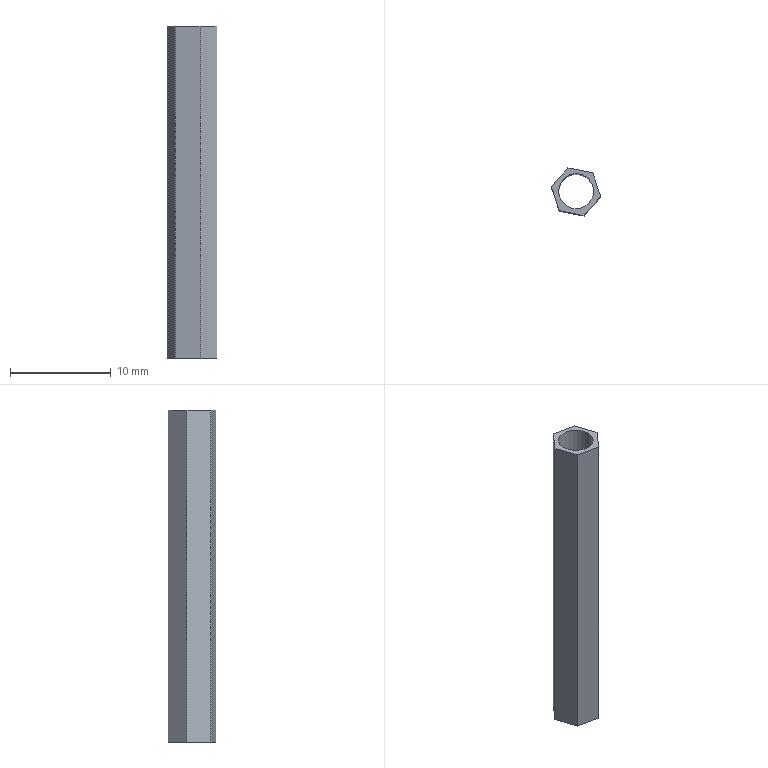Component | SolidWorks | HexStandoff-2 | 1 solid | 10 faces | box 4.92 x 4.75 x 33 mm | volume 227 mm3 | plane 8 | cylinder 2 | commonest cylinder face diameters 3.47 x2
build123d program:
from build123d import *

# Parameters (mm, degrees)
BOSS_EXTRUDE1_DEPTH     = 33
CUT_EXTRUDE1_DEPTH      = 164.264
CUT_EXTRUDE1_DEPTH_BACK = 164.264
SKETCH2_R               = 1.735


with BuildPart() as part:
    # Sketch1 → Boss-Extrude1 (new body)
    with BuildSketch(Plane.XY):
        Polygon((-154.452, -21.596), (-156.91, -22.094), (-157.708, -24.471), (-156.048, -26.351), (-153.59, -25.853), (-152.792, -23.476), align=None)
    extrude(amount=BOSS_EXTRUDE1_DEPTH)

    # Sketch2 → Cut-Extrude1 (cut, two sides: drawn at the far end of the back side and taken through both)
    with BuildSketch(Plane.XY.offset(33).offset(-CUT_EXTRUDE1_DEPTH_BACK)):
        with Locations((-155.258, -23.933)):
            Circle(SKETCH2_R)
    extrude(amount=CUT_EXTRUDE1_DEPTH + CUT_EXTRUDE1_DEPTH_BACK, mode=Mode.SUBTRACT)


solid = part.part

# Placed as in the assembly
solid = solid.moved(Location((-60.744, 0.3563, 17.5), (-180, 0, 180)))
STEP:
#1=COLOUR_RGB('',0.7922,0.8196,0.9333);
#2=FILL_AREA_STYLE_COLOUR('',#1);
#3=FILL_AREA_STYLE('',(#2));
#4=SURFACE_STYLE_FILL_AREA(#3);
#5=SURFACE_SIDE_STYLE('',(#4));
#6=SURFACE_STYLE_USAGE(.BOTH.,#5);
#7=PRESENTATION_STYLE_ASSIGNMENT((#6));
#8=CARTESIAN_POINT('',(3.789,-0.9282,0.689));
#9=VERTEX_POINT('',#8);
#10=CARTESIAN_POINT('',(3.653,-0.9282,0.689));
#11=VERTEX_POINT('',#10);
#12=CARTESIAN_POINT('',(3.721,-0.9282,0.689));
#13=DIRECTION('',(0.,0.,-1.));
#14=DIRECTION('',(-1.,0.,0.));
#15=AXIS2_PLACEMENT_3D('',#12,#13,#14);
#16=CIRCLE('',#15,0.06831);
#17=EDGE_CURVE('',#9,#11,#16,.T.);
#18=ORIENTED_EDGE('',*,*,#17,.F.);
#19=CARTESIAN_POINT('',(3.789,-0.9282,-0.6102));
#20=VERTEX_POINT('',#19);
#21=CARTESIAN_POINT('',(3.789,-0.9282,0.689));
#22=DIRECTION('',(0.,0.,-1.));
#23=VECTOR('',#22,39.37);
#24=LINE('',#21,#23);
#25=EDGE_CURVE('',#9,#20,#24,.T.);
#26=ORIENTED_EDGE('',*,*,#25,.T.);
#27=CARTESIAN_POINT('',(3.653,-0.9282,-0.6102));
#28=VERTEX_POINT('',#27);
#29=CARTESIAN_POINT('',(3.721,-0.9282,-0.6102));
#30=DIRECTION('',(0.,0.,-1.));
#31=DIRECTION('',(-1.,0.,0.));
#32=AXIS2_PLACEMENT_3D('',#29,#30,#31);
#33=CIRCLE('',#32,0.06831);
#34=EDGE_CURVE('',#20,#28,#33,.T.);
#35=ORIENTED_EDGE('',*,*,#34,.T.);
#36=CARTESIAN_POINT('',(3.653,-0.9282,0.689));
#37=DIRECTION('',(0.,0.,-1.));
#38=VECTOR('',#37,39.37);
#39=LINE('',#36,#38);
#40=EDGE_CURVE('',#11,#28,#39,.T.);
#41=ORIENTED_EDGE('',*,*,#40,.F.);
#42=EDGE_LOOP('',(#18,#26,#35,#41));
#43=FACE_OUTER_BOUND('',#42,.T.);
#44=CARTESIAN_POINT('',(3.721,-0.9282,0.689));
#45=DIRECTION('',(0.,0.,-1.));
#46=DIRECTION('',(-1.,0.,0.));
#47=AXIS2_PLACEMENT_3D('',#44,#45,#46);
#48=CYLINDRICAL_SURFACE('',#47,0.06831);
#49=ADVANCED_FACE('',(#43),#48,.F.);
#50=CARTESIAN_POINT('',(3.624,-0.9102,0.689));
#51=VERTEX_POINT('',#50);
#52=CARTESIAN_POINT('',(3.689,-0.8362,0.689));
#53=VERTEX_POINT('',#52);
#54=CARTESIAN_POINT('',(3.624,-0.9102,0.689));
#55=DIRECTION('',(0.6619,0.7496,0.));
#56=VECTOR('',#55,39.37);
#57=LINE('',#54,#56);
#58=EDGE_CURVE('',#51,#53,#57,.T.);
#59=ORIENTED_EDGE('',*,*,#58,.T.);
#60=CARTESIAN_POINT('',(3.689,-0.8362,-0.6102));
#61=VERTEX_POINT('',#60);
#62=CARTESIAN_POINT('',(3.689,-0.8362,-0.6102));
#63=DIRECTION('',(0.,0.,1.));
#64=VECTOR('',#63,39.37);
#65=LINE('',#62,#64);
#66=EDGE_CURVE('',#61,#53,#65,.T.);
#67=ORIENTED_EDGE('',*,*,#66,.F.);
#68=CARTESIAN_POINT('',(3.624,-0.9102,-0.6102));
#69=VERTEX_POINT('',#68);
#70=CARTESIAN_POINT('',(3.624,-0.9102,-0.6102));
#71=DIRECTION('',(0.6619,0.7496,0.));
#72=VECTOR('',#71,39.37);
#73=LINE('',#70,#72);
#74=EDGE_CURVE('',#69,#61,#73,.T.);
#75=ORIENTED_EDGE('',*,*,#74,.F.);
#76=CARTESIAN_POINT('',(3.624,-0.9102,-0.6102));
#77=DIRECTION('',(0.,0.,1.));
#78=VECTOR('',#77,39.37);
#79=LINE('',#76,#78);
#80=EDGE_CURVE('',#69,#51,#79,.T.);
#81=ORIENTED_EDGE('',*,*,#80,.T.);
#82=EDGE_LOOP('',(#59,#67,#75,#81));
#83=FACE_OUTER_BOUND('',#82,.T.);
#84=CARTESIAN_POINT('',(3.624,-0.9102,-0.6102));
#85=DIRECTION('',(0.7496,-0.6619,0.));
#86=DIRECTION('',(-0.6619,-0.7496,0.));
#87=AXIS2_PLACEMENT_3D('',#84,#85,#86);
#88=PLANE('',#87);
#89=ADVANCED_FACE('',(#83),#88,.F.);
#90=CARTESIAN_POINT('',(3.786,-0.8558,0.689));
#91=VERTEX_POINT('',#90);
#92=CARTESIAN_POINT('',(3.689,-0.8362,0.689));
#93=DIRECTION('',(0.9801,-0.1985,0.));
#94=VECTOR('',#93,39.37);
#95=LINE('',#92,#94);
#96=EDGE_CURVE('',#53,#91,#95,.T.);
#97=ORIENTED_EDGE('',*,*,#96,.T.);
#98=CARTESIAN_POINT('',(3.786,-0.8558,-0.6102));
#99=VERTEX_POINT('',#98);
#100=CARTESIAN_POINT('',(3.786,-0.8558,-0.6102));
#101=DIRECTION('',(0.,0.,1.));
#102=VECTOR('',#101,39.37);
#103=LINE('',#100,#102);
#104=EDGE_CURVE('',#99,#91,#103,.T.);
#105=ORIENTED_EDGE('',*,*,#104,.F.);
#106=CARTESIAN_POINT('',(3.689,-0.8362,-0.6102));
#107=DIRECTION('',(0.9801,-0.1985,0.));
#108=VECTOR('',#107,39.37);
#109=LINE('',#106,#108);
#110=EDGE_CURVE('',#61,#99,#109,.T.);
#111=ORIENTED_EDGE('',*,*,#110,.F.);
#112=ORIENTED_EDGE('',*,*,#66,.T.);
#113=EDGE_LOOP('',(#97,#105,#111,#112));
#114=FACE_OUTER_BOUND('',#113,.T.);
#115=CARTESIAN_POINT('',(3.689,-0.8362,-0.6102));
#116=DIRECTION('',(-0.1985,-0.9801,0.));
#117=DIRECTION('',(-0.9801,0.1985,0.));
#118=AXIS2_PLACEMENT_3D('',#115,#116,#117);
#119=PLANE('',#118);
#120=ADVANCED_FACE('',(#114),#119,.F.);
#121=CARTESIAN_POINT('',(3.817,-0.9494,0.689));
#122=VERTEX_POINT('',#121);
#123=CARTESIAN_POINT('',(3.786,-0.8558,0.689));
#124=DIRECTION('',(0.3182,-0.948,0.));
#125=VECTOR('',#124,39.37);
#126=LINE('',#123,#125);
#127=EDGE_CURVE('',#91,#122,#126,.T.);
#128=ORIENTED_EDGE('',*,*,#127,.T.);
#129=CARTESIAN_POINT('',(3.817,-0.9494,-0.6102));
#130=VERTEX_POINT('',#129);
#131=CARTESIAN_POINT('',(3.817,-0.9494,-0.6102));
#132=DIRECTION('',(0.,0.,1.));
#133=VECTOR('',#132,39.37);
#134=LINE('',#131,#133);
#135=EDGE_CURVE('',#130,#122,#134,.T.);
#136=ORIENTED_EDGE('',*,*,#135,.F.);
#137=CARTESIAN_POINT('',(3.786,-0.8558,-0.6102));
#138=DIRECTION('',(0.3182,-0.948,0.));
#139=VECTOR('',#138,39.37);
#140=LINE('',#137,#139);
#141=EDGE_CURVE('',#99,#130,#140,.T.);
#142=ORIENTED_EDGE('',*,*,#141,.F.);
#143=ORIENTED_EDGE('',*,*,#104,.T.);
#144=EDGE_LOOP('',(#128,#136,#142,#143));
#145=FACE_OUTER_BOUND('',#144,.T.);
#146=CARTESIAN_POINT('',(3.786,-0.8558,-0.6102));
#147=DIRECTION('',(-0.948,-0.3182,0.));
#148=DIRECTION('',(-0.3182,0.948,0.));
#149=AXIS2_PLACEMENT_3D('',#146,#147,#148);
#150=PLANE('',#149);
#151=ADVANCED_FACE('',(#145),#150,.F.);
#152=CARTESIAN_POINT('',(3.752,-1.023,0.689));
#153=VERTEX_POINT('',#152);
#154=CARTESIAN_POINT('',(3.817,-0.9494,0.689));
#155=DIRECTION('',(-0.6619,-0.7496,0.));
#156=VECTOR('',#155,39.37);
#157=LINE('',#154,#156);
#158=EDGE_CURVE('',#122,#153,#157,.T.);
#159=ORIENTED_EDGE('',*,*,#158,.T.);
#160=CARTESIAN_POINT('',(3.752,-1.023,-0.6102));
#161=VERTEX_POINT('',#160);
#162=CARTESIAN_POINT('',(3.752,-1.023,-0.6102));
#163=DIRECTION('',(0.,0.,1.));
#164=VECTOR('',#163,39.37);
#165=LINE('',#162,#164);
#166=EDGE_CURVE('',#161,#153,#165,.T.);
#167=ORIENTED_EDGE('',*,*,#166,.F.);
#168=CARTESIAN_POINT('',(3.817,-0.9494,-0.6102));
#169=DIRECTION('',(-0.6619,-0.7496,0.));
#170=VECTOR('',#169,39.37);
#171=LINE('',#168,#170);
#172=EDGE_CURVE('',#130,#161,#171,.T.);
#173=ORIENTED_EDGE('',*,*,#172,.F.);
#174=ORIENTED_EDGE('',*,*,#135,.T.);
#175=EDGE_LOOP('',(#159,#167,#173,#174));
#176=FACE_OUTER_BOUND('',#175,.T.);
#177=CARTESIAN_POINT('',(3.817,-0.9494,-0.6102));
#178=DIRECTION('',(-0.7496,0.6619,0.));
#179=DIRECTION('',(0.6619,0.7496,0.));
#180=AXIS2_PLACEMENT_3D('',#177,#178,#179);
#181=PLANE('',#180);
#182=ADVANCED_FACE('',(#176),#181,.F.);
#183=CARTESIAN_POINT('',(3.655,-1.004,0.689));
#184=VERTEX_POINT('',#183);
#185=CARTESIAN_POINT('',(3.752,-1.023,0.689));
#186=DIRECTION('',(-0.9801,0.1985,0.));
#187=VECTOR('',#186,39.37);
#188=LINE('',#185,#187);
#189=EDGE_CURVE('',#153,#184,#188,.T.);
#190=ORIENTED_EDGE('',*,*,#189,.T.);
#191=CARTESIAN_POINT('',(3.655,-1.004,-0.6102));
#192=VERTEX_POINT('',#191);
#193=CARTESIAN_POINT('',(3.655,-1.004,-0.6102));
#194=DIRECTION('',(0.,0.,1.));
#195=VECTOR('',#194,39.37);
#196=LINE('',#193,#195);
#197=EDGE_CURVE('',#192,#184,#196,.T.);
#198=ORIENTED_EDGE('',*,*,#197,.F.);
#199=CARTESIAN_POINT('',(3.752,-1.023,-0.6102));
#200=DIRECTION('',(-0.9801,0.1985,0.));
#201=VECTOR('',#200,39.37);
#202=LINE('',#199,#201);
#203=EDGE_CURVE('',#161,#192,#202,.T.);
#204=ORIENTED_EDGE('',*,*,#203,.F.);
#205=ORIENTED_EDGE('',*,*,#166,.T.);
#206=EDGE_LOOP('',(#190,#198,#204,#205));
#207=FACE_OUTER_BOUND('',#206,.T.);
#208=CARTESIAN_POINT('',(3.752,-1.023,-0.6102));
#209=DIRECTION('',(0.1985,0.9801,0.));
#210=DIRECTION('',(0.9801,-0.1985,0.));
#211=AXIS2_PLACEMENT_3D('',#208,#209,#210);
#212=PLANE('',#211);
#213=ADVANCED_FACE('',(#207),#212,.F.);
#214=CARTESIAN_POINT('',(3.655,-1.004,0.689));
#215=DIRECTION('',(-0.3182,0.948,0.));
#216=VECTOR('',#215,39.37);
#217=LINE('',#214,#216);
#218=EDGE_CURVE('',#184,#51,#217,.T.);
#219=ORIENTED_EDGE('',*,*,#218,.T.);
#220=ORIENTED_EDGE('',*,*,#80,.F.);
#221=CARTESIAN_POINT('',(3.655,-1.004,-0.6102));
#222=DIRECTION('',(-0.3182,0.948,0.));
#223=VECTOR('',#222,39.37);
#224=LINE('',#221,#223);
#225=EDGE_CURVE('',#192,#69,#224,.T.);
#226=ORIENTED_EDGE('',*,*,#225,.F.);
#227=ORIENTED_EDGE('',*,*,#197,.T.);
#228=EDGE_LOOP('',(#219,#220,#226,#227));
#229=FACE_OUTER_BOUND('',#228,.T.);
#230=CARTESIAN_POINT('',(3.655,-1.004,-0.6102));
#231=DIRECTION('',(0.948,0.3182,0.));
#232=DIRECTION('',(0.3182,-0.948,0.));
#233=AXIS2_PLACEMENT_3D('',#230,#231,#232);
#234=PLANE('',#233);
#235=ADVANCED_FACE('',(#229),#234,.F.);
#236=CARTESIAN_POINT('',(3.721,-0.9282,-0.6102));
#237=DIRECTION('',(0.,0.,-1.));
#238=DIRECTION('',(-1.,0.,0.));
#239=AXIS2_PLACEMENT_3D('',#236,#237,#238);
#240=CIRCLE('',#239,0.06831);
#241=EDGE_CURVE('',#28,#20,#240,.T.);
#242=ORIENTED_EDGE('',*,*,#241,.F.);
#243=ORIENTED_EDGE('',*,*,#34,.F.);
#244=EDGE_LOOP('',(#242,#243));
#245=FACE_BOUND('',#244,.T.);
#246=ORIENTED_EDGE('',*,*,#74,.T.);
#247=ORIENTED_EDGE('',*,*,#110,.T.);
#248=ORIENTED_EDGE('',*,*,#141,.T.);
#249=ORIENTED_EDGE('',*,*,#172,.T.);
#250=ORIENTED_EDGE('',*,*,#203,.T.);
#251=ORIENTED_EDGE('',*,*,#225,.T.);
#252=EDGE_LOOP('',(#246,#247,#248,#249,#250,#251));
#253=FACE_OUTER_BOUND('',#252,.T.);
#254=CARTESIAN_POINT('',(-2.391,0.01403,-0.6102));
#255=DIRECTION('',(0.,0.,-1.));
#256=DIRECTION('',(-1.,0.,0.));
#257=AXIS2_PLACEMENT_3D('',#254,#255,#256);
#258=PLANE('',#257);
#259=ADVANCED_FACE('',(#245,#253),#258,.T.);
#260=CARTESIAN_POINT('',(3.721,-0.9282,0.689));
#261=DIRECTION('',(0.,0.,-1.));
#262=DIRECTION('',(-1.,0.,0.));
#263=AXIS2_PLACEMENT_3D('',#260,#261,#262);
#264=CIRCLE('',#263,0.06831);
#265=EDGE_CURVE('',#11,#9,#264,.T.);
#266=ORIENTED_EDGE('',*,*,#265,.T.);
#267=ORIENTED_EDGE('',*,*,#17,.T.);
#268=EDGE_LOOP('',(#266,#267));
#269=FACE_BOUND('',#268,.T.);
#270=ORIENTED_EDGE('',*,*,#58,.F.);
#271=ORIENTED_EDGE('',*,*,#218,.F.);
#272=ORIENTED_EDGE('',*,*,#189,.F.);
#273=ORIENTED_EDGE('',*,*,#158,.F.);
#274=ORIENTED_EDGE('',*,*,#127,.F.);
#275=ORIENTED_EDGE('',*,*,#96,.F.);
#276=EDGE_LOOP('',(#270,#271,#272,#273,#274,#275));
#277=FACE_OUTER_BOUND('',#276,.T.);
#278=CARTESIAN_POINT('',(-2.391,0.01403,0.689));
#279=DIRECTION('',(0.,0.,-1.));
#280=DIRECTION('',(-1.,0.,0.));
#281=AXIS2_PLACEMENT_3D('',#278,#279,#280);
#282=PLANE('',#281);
#283=ADVANCED_FACE('',(#269,#277),#282,.F.);
#284=ORIENTED_EDGE('',*,*,#25,.F.);
#285=ORIENTED_EDGE('',*,*,#265,.F.);
#286=ORIENTED_EDGE('',*,*,#40,.T.);
#287=ORIENTED_EDGE('',*,*,#241,.T.);
#288=EDGE_LOOP('',(#284,#285,#286,#287));
#289=FACE_OUTER_BOUND('',#288,.T.);
#290=CARTESIAN_POINT('',(3.721,-0.9282,0.689));
#291=DIRECTION('',(0.,0.,-1.));
#292=DIRECTION('',(-1.,0.,0.));
#293=AXIS2_PLACEMENT_3D('',#290,#291,#292);
#294=CYLINDRICAL_SURFACE('',#293,0.06831);
#295=ADVANCED_FACE('',(#289),#294,.F.);
#296=CLOSED_SHELL('',(#49,#89,#120,#151,#182,#213,#235,#259,#283,#295));
#297=MANIFOLD_SOLID_BREP('',#296);
#298=STYLED_ITEM('',(#7),#297);
#299=(LENGTH_UNIT()NAMED_UNIT(*)SI_UNIT($,.METRE.));
#300=LENGTH_MEASURE_WITH_UNIT(LENGTH_MEASURE(0.0254),#299);
#301=DIMENSIONAL_EXPONENTS(1.,0.,0.,0.,0.,0.,0.);
#302=(CONVERSION_BASED_UNIT('',#300)LENGTH_UNIT()NAMED_UNIT(#301));
#303=UNCERTAINTY_MEASURE_WITH_UNIT(LENGTH_MEASURE(0.00001),#302,'','');
#304=(NAMED_UNIT(*)PLANE_ANGLE_UNIT()SI_UNIT($,.RADIAN.));
#305=(NAMED_UNIT(*)SI_UNIT($,.STERADIAN.)SOLID_ANGLE_UNIT());
#306=(GEOMETRIC_REPRESENTATION_CONTEXT(3)GLOBAL_UNCERTAINTY_ASSIGNED_CONTEXT((#303))GLOBAL_UNIT_ASSIGNED_CONTEXT((#302,#304,#305))REPRESENTATION_CONTEXT('',''));
#307=MECHANICAL_DESIGN_GEOMETRIC_PRESENTATION_REPRESENTATION('',(#298),#306);
#308=CARTESIAN_POINT('',(0.,0.,0.));
#309=DIRECTION('',(0.,0.,1.));
#310=DIRECTION('',(1.,0.,0.));
#311=AXIS2_PLACEMENT_3D('',#308,#309,#310);
#312=(LENGTH_UNIT()NAMED_UNIT(*)SI_UNIT($,.METRE.));
#313=LENGTH_MEASURE_WITH_UNIT(LENGTH_MEASURE(0.0254),#312);
#314=DIMENSIONAL_EXPONENTS(1.,0.,0.,0.,0.,0.,0.);
#315=(CONVERSION_BASED_UNIT('',#313)LENGTH_UNIT()NAMED_UNIT(#314));
#316=UNCERTAINTY_MEASURE_WITH_UNIT(LENGTH_MEASURE(0.00001),#315,'','');
#317=(NAMED_UNIT(*)PLANE_ANGLE_UNIT()SI_UNIT($,.RADIAN.));
#318=(NAMED_UNIT(*)SI_UNIT($,.STERADIAN.)SOLID_ANGLE_UNIT());
#319=(GEOMETRIC_REPRESENTATION_CONTEXT(3)GLOBAL_UNCERTAINTY_ASSIGNED_CONTEXT((#316))GLOBAL_UNIT_ASSIGNED_CONTEXT((#315,#317,#318))REPRESENTATION_CONTEXT('',''));
#320=ADVANCED_BREP_SHAPE_REPRESENTATION('',(#297,#311),#319);
#321=PRESENTATION_LAYER_ASSIGNMENT('','',(#298));